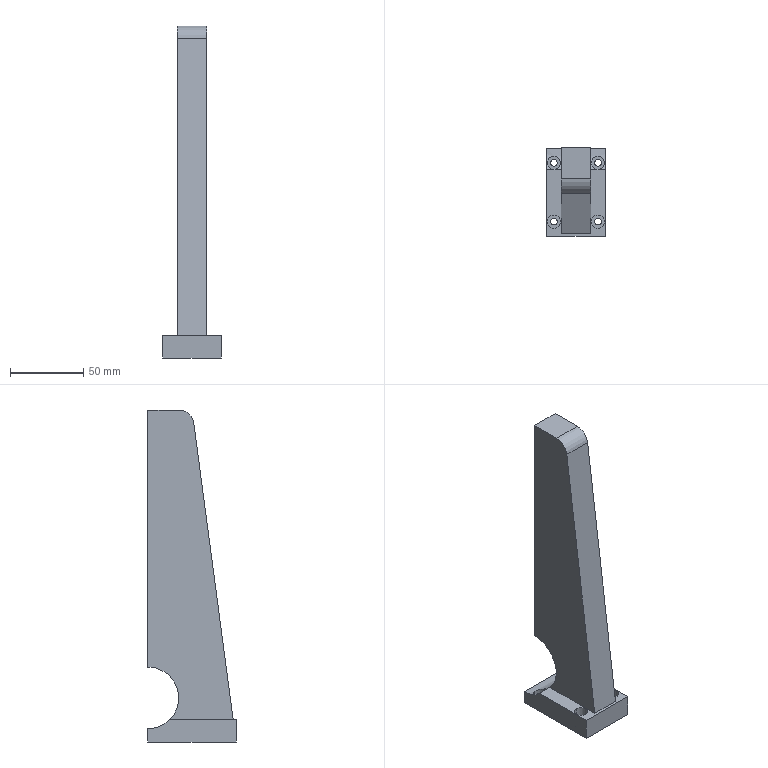CAM job | Mastercam | mm | 1 operations | part box 40 x 60 x 226
1. Drill/Counterbore | 14 - 8 平铣刀